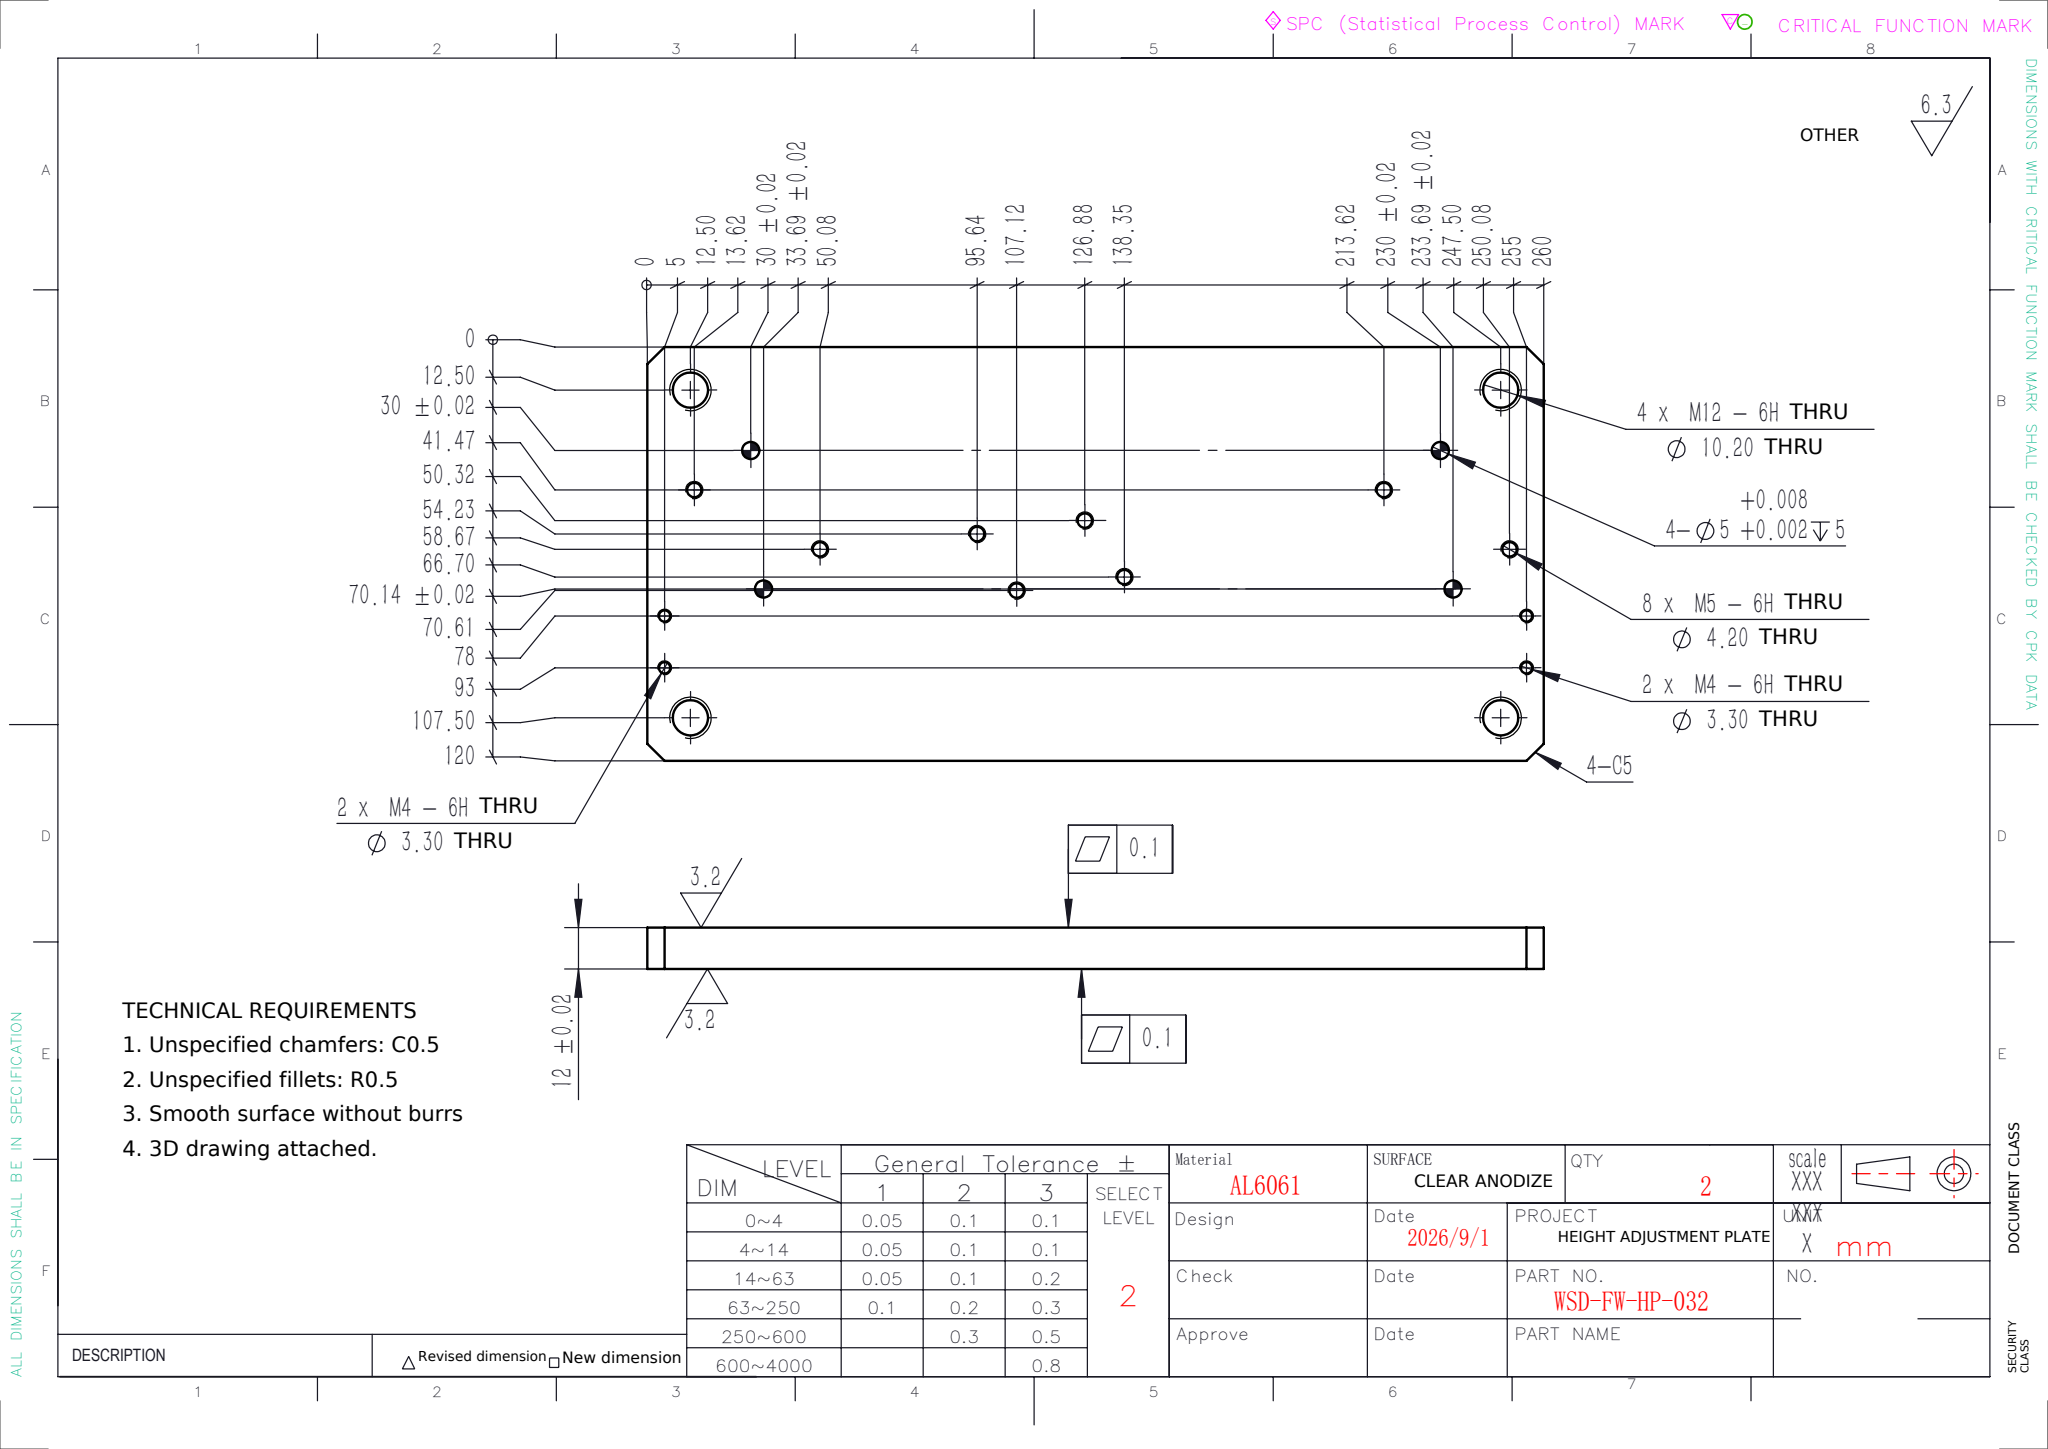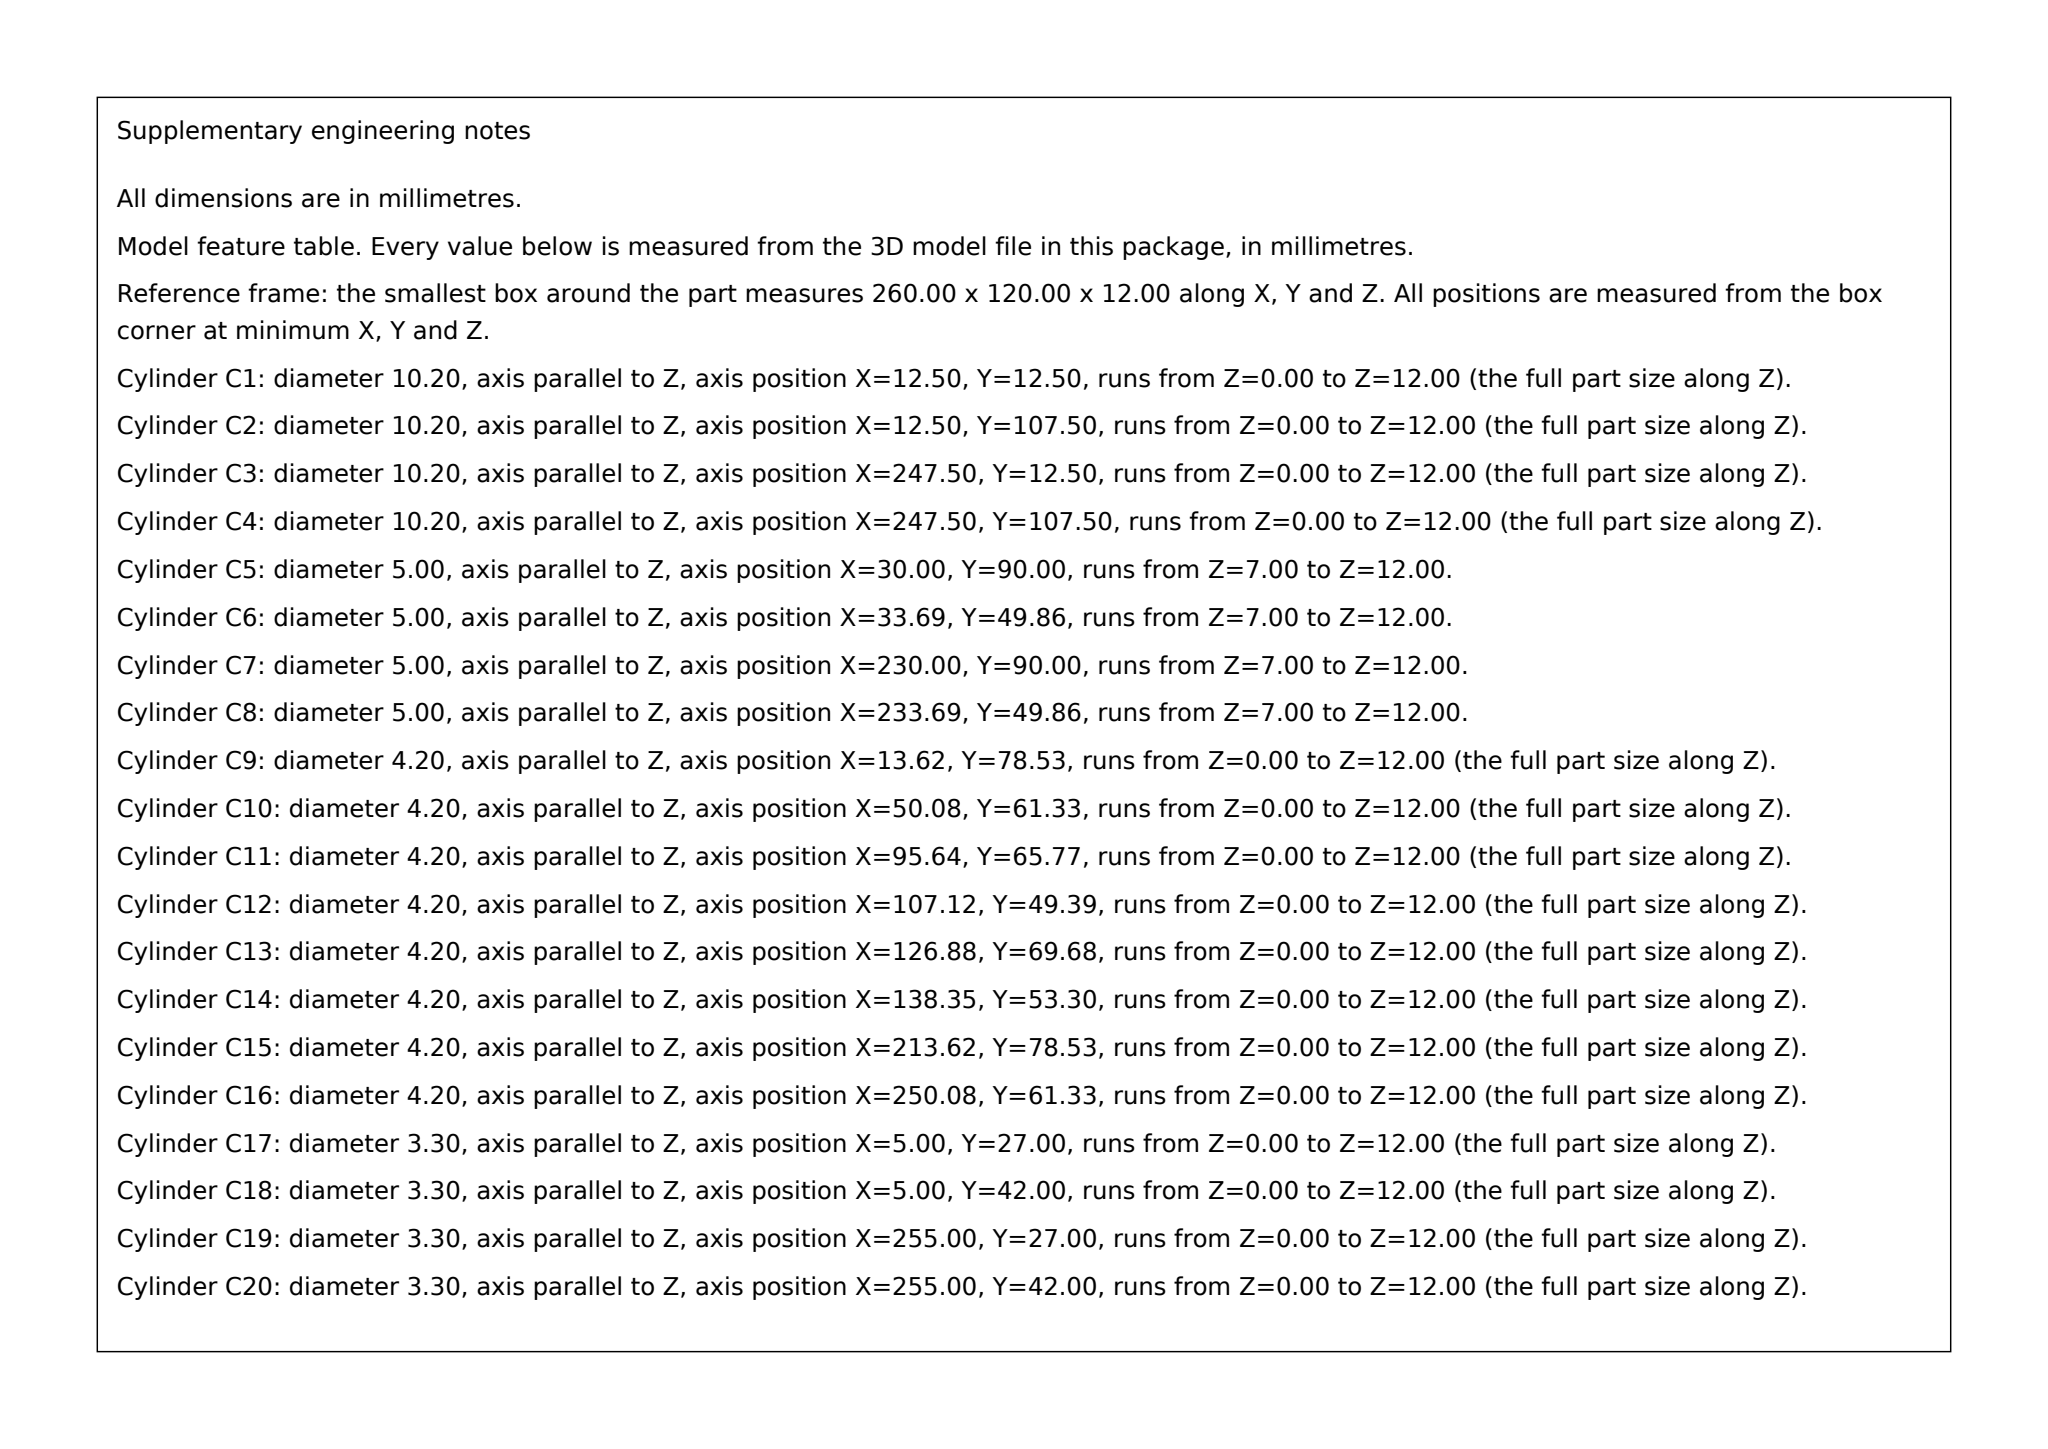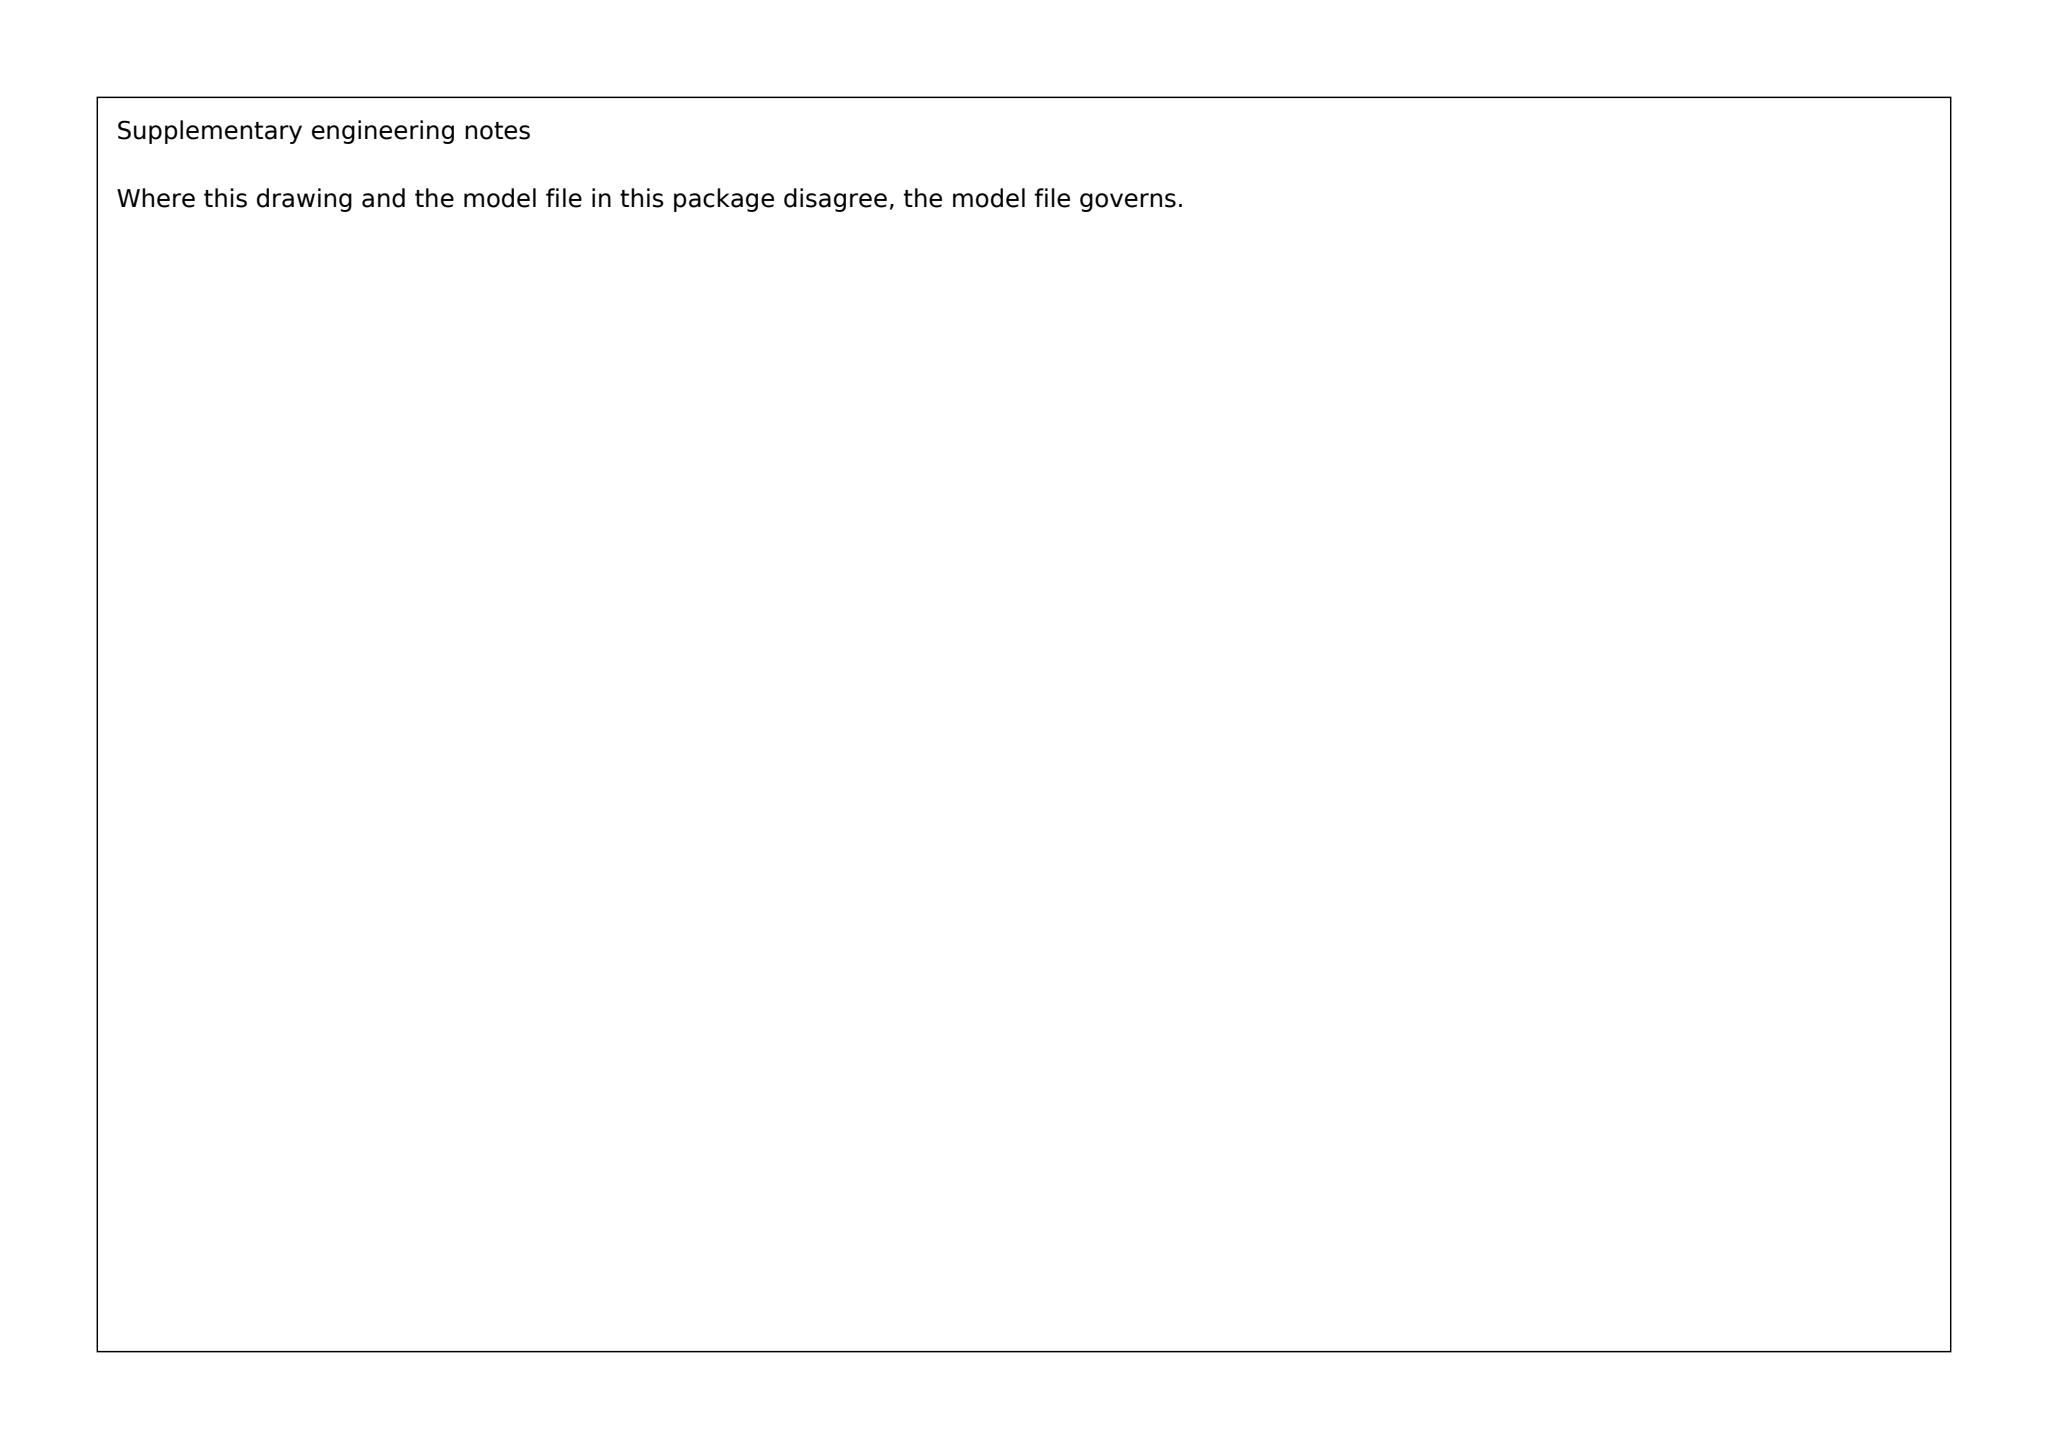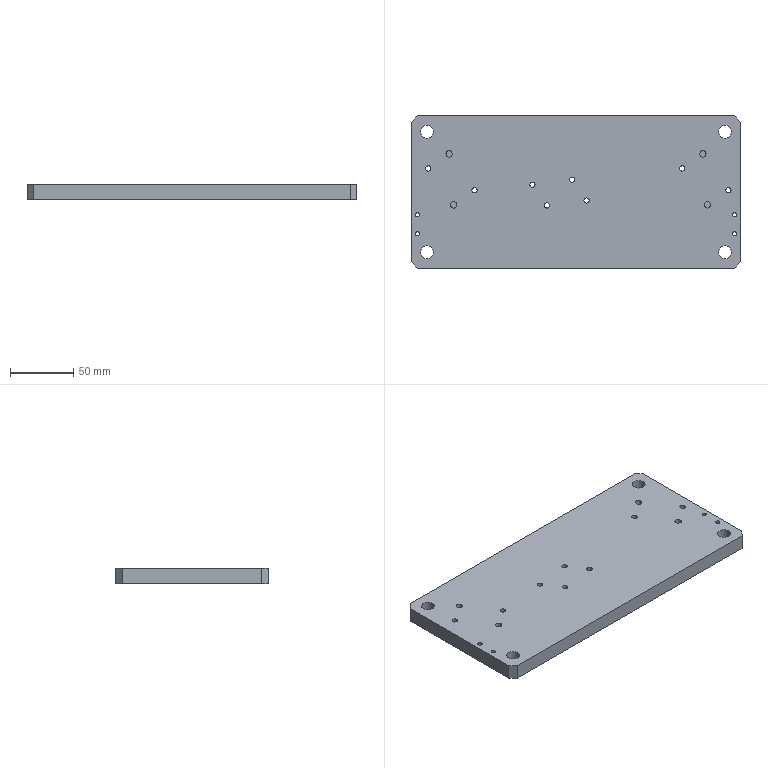Part | SolidWorks | mm | 1 solid | 54 faces | box 260 x 120 x 12 mm | volume 367745 mm3 | cylinder 40 | plane 14 | commonest cylinder face diameters 4.2 x16 5 x8 3.3 x8 10.2 x8
build123d program:
from build123d import *

# Parameters (mm, degrees)
SKETCH1_W             = 260
SKETCH1_H             = 120
BOSS_EXTRUDE1_DEPTH   = 12
M12_TAPPED_HOLE1_D    = 10.2
CHAMFER1_SIZE         = 5
M4_TAPPED_HOLE1_D     = 3.3
M4_TAPPED_HOLE2_D     = 3.3
SKETCH12_R            = 2.5
CUT_EXTRUDE1_DEPTH    = 5
M5_TAPPED_HOLE1_D     = 4.2
M5_TAPPED_HOLE2_D     = 4.2
M5_TAPPED_HOLE2_DEPTH = 12.4
M5_TAPPED_HOLE2_TIP   = 1.262


with BuildPart() as part:
    # Sketch1 → Boss-Extrude1 (new body)
    with BuildSketch(Plane.XY):
        Rectangle(SKETCH1_W, SKETCH1_H)
    extrude(amount=BOSS_EXTRUDE1_DEPTH)

    # M12 Tapped Hole1 (through all)
    with Locations(Plane.XY.offset(12)):
        with Locations((-117.5, 47.5), (117.5, 47.5), (117.5, -47.5), (-117.5, -47.5)):
            Hole(M12_TAPPED_HOLE1_D / 2)

    # Chamfer1
    chamfer1_edges = [part.edges().sort_by_distance(p)[0] for p in [
        (130, -60, 6),
        (-130, -60, 6),
        (-130, 60, 6),
        (130, 60, 6),
    ]]
    chamfer(chamfer1_edges, length=CHAMFER1_SIZE)

    # M4 Tapped Hole1 (through all)
    with Locations(Plane.XY.offset(12)):
        with Locations((125, -18), (125, -33)):
            Hole(M4_TAPPED_HOLE1_D / 2)

    # M4 Tapped Hole2 (through all)
    with Locations(Plane.XY.offset(12)):
        with Locations((-125, -18), (-125, -33)):
            Hole(M4_TAPPED_HOLE2_D / 2)

    # Sketch12 → Cut-Extrude1 (cut)
    with BuildSketch(Plane.XY.offset(12)):
        with Locations((100, 30)):
            Circle(SKETCH12_R)
        with Locations((103.692, -10.142)):
            Circle(SKETCH12_R)
        with Locations((-96.308, -10.142)):
            Circle(SKETCH12_R)
        with Locations((-100, 30)):
            Circle(SKETCH12_R)
    extrude(amount=-CUT_EXTRUDE1_DEPTH, mode=Mode.SUBTRACT)

    # M5 Tapped Hole1 (through all)
    with Locations(Plane.XY.offset(12)):
        with Locations((-79.925, 1.33), (-116.383, 18.528), (83.617, 18.528), (120.075, 1.33)):
            Hole(M5_TAPPED_HOLE1_D / 2)

    # M5 Tapped Hole2
    with Locations(Plane.XY.offset(12)):
        with Locations((-22.884, -10.613), (-34.356, 5.77), (-3.118, 9.679), (8.354, -6.704)):
            Hole(M5_TAPPED_HOLE2_D / 2, depth=M5_TAPPED_HOLE2_DEPTH)
            with Locations((0, 0, -(M5_TAPPED_HOLE2_DEPTH + M5_TAPPED_HOLE2_TIP / 2))):  # 118° drill point
                Cone(0, M5_TAPPED_HOLE2_D / 2, M5_TAPPED_HOLE2_TIP, mode=Mode.SUBTRACT)


solid = part.part